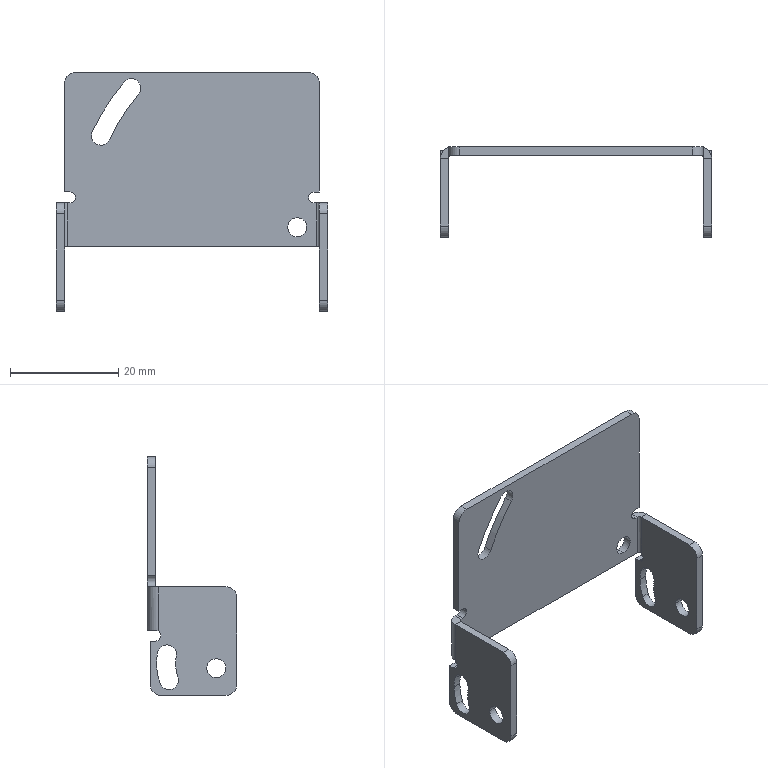Component | SolidWorks | F01AE00111-A5219-1 | 1 solid | 69 faces | volume 2992 mm3 | cylinder 39 | plane 28 | spline 2 | commonest cylinder face diameters 3.5 x13 4 x10 22 x4 15 x4 2 x4 1 x2 76.381 x1 83.381 x1